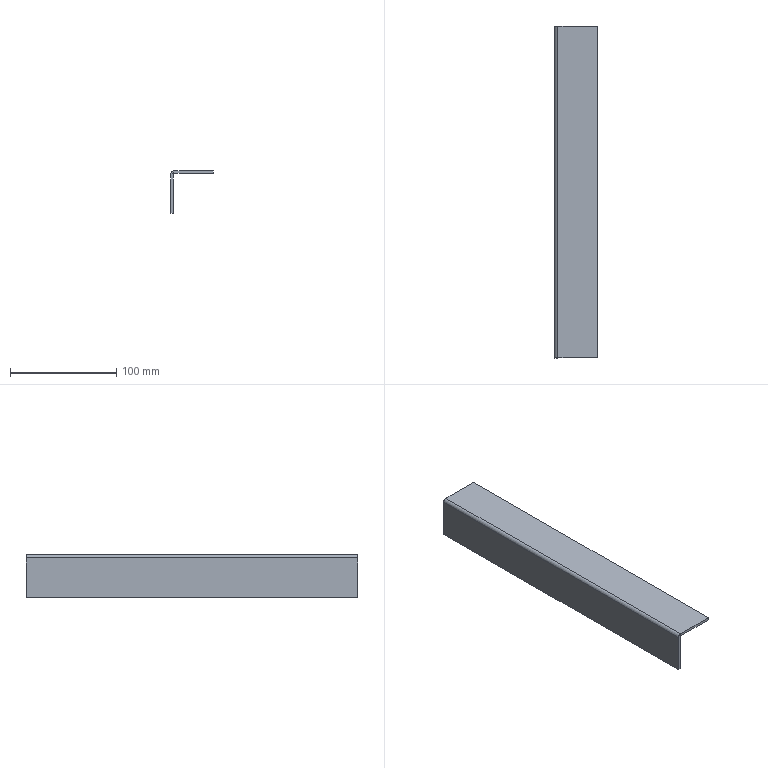Component | SolidWorks | BottomFrameAssembly2-1_CabinetDepthBeam-2 | 1 solid | 14 faces | box 40 x 313 x 40 mm | volume 60056 mm3 | plane 12 | cylinder 2 | commonest cylinder face diameters 1 x1 6 x1
STEP:
#1=CARTESIAN_POINT('',(-5.573,-6.388,66.81));
#2=VERTEX_POINT('',#1);
#3=CARTESIAN_POINT('',(-5.672,-6.388,66.81));
#4=VERTEX_POINT('',#3);
#5=CARTESIAN_POINT('',(-5.573,-6.388,66.81));
#6=DIRECTION('',(-1.,-0.,0.));
#7=VECTOR('',#6,39.37);
#8=LINE('',#5,#7);
#9=EDGE_CURVE('',#2,#4,#8,.T.);
#10=ORIENTED_EDGE('',*,*,#9,.F.);
#11=CARTESIAN_POINT('',(-5.554,-6.388,66.83));
#12=VERTEX_POINT('',#11);
#13=CARTESIAN_POINT('',(-5.554,-6.388,66.81));
#14=DIRECTION('',(0.,-1.,0.));
#15=DIRECTION('',(1.,0.,0.));
#16=AXIS2_PLACEMENT_3D('',#13,#14,#15);
#17=CIRCLE('',#16,0.01969);
#18=EDGE_CURVE('',#12,#2,#17,.T.);
#19=ORIENTED_EDGE('',*,*,#18,.F.);
#20=CARTESIAN_POINT('',(-5.554,-6.388,66.928));
#21=VERTEX_POINT('',#20);
#22=CARTESIAN_POINT('',(-5.554,-6.388,66.928));
#23=DIRECTION('',(0.,-0.,-1.));
#24=VECTOR('',#23,39.37);
#25=LINE('',#22,#24);
#26=EDGE_CURVE('',#21,#12,#25,.T.);
#27=ORIENTED_EDGE('',*,*,#26,.F.);
#28=CARTESIAN_POINT('',(-5.554,-6.388,66.81));
#29=DIRECTION('',(0.,-1.,0.));
#30=DIRECTION('',(-1.,-0.,0.));
#31=AXIS2_PLACEMENT_3D('',#28,#29,#30);
#32=CIRCLE('',#31,0.1181);
#33=EDGE_CURVE('',#21,#4,#32,.T.);
#34=ORIENTED_EDGE('',*,*,#33,.T.);
#35=EDGE_LOOP('',(#10,#19,#27,#34));
#36=FACE_OUTER_BOUND('',#35,.T.);
#37=CARTESIAN_POINT('',(-5.573,-6.388,66.81));
#38=DIRECTION('',(0.,-1.,0.));
#39=DIRECTION('',(-1.,-0.,0.));
#40=AXIS2_PLACEMENT_3D('',#37,#38,#39);
#41=PLANE('',#40);
#42=ADVANCED_FACE('',(#36),#41,.T.);
#43=CARTESIAN_POINT('',(-5.573,-6.388,65.354));
#44=VERTEX_POINT('',#43);
#45=CARTESIAN_POINT('',(-5.573,-6.388,66.83));
#46=DIRECTION('',(0.,-0.,-1.));
#47=VECTOR('',#46,39.37);
#48=LINE('',#45,#47);
#49=EDGE_CURVE('',#2,#44,#48,.T.);
#50=ORIENTED_EDGE('',*,*,#49,.F.);
#51=ORIENTED_EDGE('',*,*,#9,.T.);
#52=CARTESIAN_POINT('',(-5.672,-6.388,65.354));
#53=VERTEX_POINT('',#52);
#54=CARTESIAN_POINT('',(-5.672,-6.388,66.83));
#55=DIRECTION('',(0.,-0.,-1.));
#56=VECTOR('',#55,39.37);
#57=LINE('',#54,#56);
#58=EDGE_CURVE('',#4,#53,#57,.T.);
#59=ORIENTED_EDGE('',*,*,#58,.T.);
#60=CARTESIAN_POINT('',(-5.573,-6.388,65.354));
#61=DIRECTION('',(-1.,-0.,0.));
#62=VECTOR('',#61,39.37);
#63=LINE('',#60,#62);
#64=EDGE_CURVE('',#44,#53,#63,.T.);
#65=ORIENTED_EDGE('',*,*,#64,.F.);
#66=EDGE_LOOP('',(#50,#51,#59,#65));
#67=FACE_OUTER_BOUND('',#66,.T.);
#68=CARTESIAN_POINT('',(-5.554,-6.388,66.928));
#69=DIRECTION('',(0.,-1.,0.));
#70=DIRECTION('',(-1.,-0.,0.));
#71=AXIS2_PLACEMENT_3D('',#68,#69,#70);
#72=PLANE('',#71);
#73=ADVANCED_FACE('',(#67),#72,.T.);
#74=CARTESIAN_POINT('',(-5.554,5.935,66.83));
#75=VERTEX_POINT('',#74);
#76=CARTESIAN_POINT('',(-5.554,5.935,66.928));
#77=VERTEX_POINT('',#76);
#78=CARTESIAN_POINT('',(-5.554,5.935,66.83));
#79=DIRECTION('',(-0.,0.,1.));
#80=VECTOR('',#79,39.37);
#81=LINE('',#78,#80);
#82=EDGE_CURVE('',#75,#77,#81,.T.);
#83=ORIENTED_EDGE('',*,*,#82,.F.);
#84=CARTESIAN_POINT('',(-5.573,5.935,66.81));
#85=VERTEX_POINT('',#84);
#86=CARTESIAN_POINT('',(-5.554,5.935,66.81));
#87=DIRECTION('',(0.,-1.,0.));
#88=DIRECTION('',(1.,0.,0.));
#89=AXIS2_PLACEMENT_3D('',#86,#87,#88);
#90=CIRCLE('',#89,0.01969);
#91=EDGE_CURVE('',#75,#85,#90,.T.);
#92=ORIENTED_EDGE('',*,*,#91,.T.);
#93=CARTESIAN_POINT('',(-5.672,5.935,66.81));
#94=VERTEX_POINT('',#93);
#95=CARTESIAN_POINT('',(-5.672,5.935,66.81));
#96=DIRECTION('',(1.,0.,-0.));
#97=VECTOR('',#96,39.37);
#98=LINE('',#95,#97);
#99=EDGE_CURVE('',#94,#85,#98,.T.);
#100=ORIENTED_EDGE('',*,*,#99,.F.);
#101=CARTESIAN_POINT('',(-5.554,5.935,66.81));
#102=DIRECTION('',(0.,-1.,0.));
#103=DIRECTION('',(-1.,-0.,0.));
#104=AXIS2_PLACEMENT_3D('',#101,#102,#103);
#105=CIRCLE('',#104,0.1181);
#106=EDGE_CURVE('',#77,#94,#105,.T.);
#107=ORIENTED_EDGE('',*,*,#106,.F.);
#108=EDGE_LOOP('',(#83,#92,#100,#107));
#109=FACE_OUTER_BOUND('',#108,.T.);
#110=CARTESIAN_POINT('',(-5.554,5.935,66.83));
#111=DIRECTION('',(-0.,1.,-0.));
#112=DIRECTION('',(1.,0.,-0.));
#113=AXIS2_PLACEMENT_3D('',#110,#111,#112);
#114=PLANE('',#113);
#115=ADVANCED_FACE('',(#109),#114,.T.);
#116=CARTESIAN_POINT('',(-4.097,5.935,66.83));
#117=VERTEX_POINT('',#116);
#118=CARTESIAN_POINT('',(-4.097,5.935,66.83));
#119=DIRECTION('',(-1.,-0.,0.));
#120=VECTOR('',#119,39.37);
#121=LINE('',#118,#120);
#122=EDGE_CURVE('',#117,#75,#121,.T.);
#123=ORIENTED_EDGE('',*,*,#122,.T.);
#124=ORIENTED_EDGE('',*,*,#82,.T.);
#125=CARTESIAN_POINT('',(-4.097,5.935,66.928));
#126=VERTEX_POINT('',#125);
#127=CARTESIAN_POINT('',(-4.097,5.935,66.928));
#128=DIRECTION('',(-1.,-0.,0.));
#129=VECTOR('',#128,39.37);
#130=LINE('',#127,#129);
#131=EDGE_CURVE('',#126,#77,#130,.T.);
#132=ORIENTED_EDGE('',*,*,#131,.F.);
#133=CARTESIAN_POINT('',(-4.097,5.935,66.928));
#134=DIRECTION('',(0.,-0.,-1.));
#135=VECTOR('',#134,39.37);
#136=LINE('',#133,#135);
#137=EDGE_CURVE('',#126,#117,#136,.T.);
#138=ORIENTED_EDGE('',*,*,#137,.T.);
#139=EDGE_LOOP('',(#123,#124,#132,#138));
#140=FACE_OUTER_BOUND('',#139,.T.);
#141=CARTESIAN_POINT('',(-5.672,5.935,66.81));
#142=DIRECTION('',(-0.,1.,-0.));
#143=DIRECTION('',(1.,0.,-0.));
#144=AXIS2_PLACEMENT_3D('',#141,#142,#143);
#145=PLANE('',#144);
#146=ADVANCED_FACE('',(#140),#145,.T.);
#147=CARTESIAN_POINT('',(-5.672,5.935,65.354));
#148=VERTEX_POINT('',#147);
#149=CARTESIAN_POINT('',(-5.672,5.935,66.83));
#150=DIRECTION('',(0.,-0.,-1.));
#151=VECTOR('',#150,39.37);
#152=LINE('',#149,#151);
#153=EDGE_CURVE('',#94,#148,#152,.T.);
#154=ORIENTED_EDGE('',*,*,#153,.T.);
#155=CARTESIAN_POINT('',(-5.672,-6.388,65.354));
#156=DIRECTION('',(-0.,1.,-0.));
#157=VECTOR('',#156,39.37);
#158=LINE('',#155,#157);
#159=EDGE_CURVE('',#53,#148,#158,.T.);
#160=ORIENTED_EDGE('',*,*,#159,.F.);
#161=ORIENTED_EDGE('',*,*,#58,.F.);
#162=CARTESIAN_POINT('',(-5.672,-6.388,66.81));
#163=DIRECTION('',(-0.,1.,-0.));
#164=VECTOR('',#163,39.37);
#165=LINE('',#162,#164);
#166=EDGE_CURVE('',#4,#94,#165,.T.);
#167=ORIENTED_EDGE('',*,*,#166,.T.);
#168=EDGE_LOOP('',(#154,#160,#161,#167));
#169=FACE_OUTER_BOUND('',#168,.T.);
#170=CARTESIAN_POINT('',(-5.672,-6.388,66.83));
#171=DIRECTION('',(1.,0.,-0.));
#172=DIRECTION('',(0.,-1.,0.));
#173=AXIS2_PLACEMENT_3D('',#170,#171,#172);
#174=PLANE('',#173);
#175=ADVANCED_FACE('',(#169),#174,.F.);
#176=CARTESIAN_POINT('',(-5.573,5.935,65.354));
#177=VERTEX_POINT('',#176);
#178=CARTESIAN_POINT('',(-5.573,5.935,65.354));
#179=DIRECTION('',(-1.,-0.,0.));
#180=VECTOR('',#179,39.37);
#181=LINE('',#178,#180);
#182=EDGE_CURVE('',#177,#148,#181,.T.);
#183=ORIENTED_EDGE('',*,*,#182,.F.);
#184=CARTESIAN_POINT('',(-5.573,-6.388,65.354));
#185=DIRECTION('',(-0.,1.,-0.));
#186=VECTOR('',#185,39.37);
#187=LINE('',#184,#186);
#188=EDGE_CURVE('',#44,#177,#187,.T.);
#189=ORIENTED_EDGE('',*,*,#188,.F.);
#190=ORIENTED_EDGE('',*,*,#64,.T.);
#191=ORIENTED_EDGE('',*,*,#159,.T.);
#192=EDGE_LOOP('',(#183,#189,#190,#191));
#193=FACE_OUTER_BOUND('',#192,.T.);
#194=CARTESIAN_POINT('',(-5.573,-6.388,65.354));
#195=DIRECTION('',(0.,-0.,-1.));
#196=DIRECTION('',(0.,-1.,0.));
#197=AXIS2_PLACEMENT_3D('',#194,#195,#196);
#198=PLANE('',#197);
#199=ADVANCED_FACE('',(#193),#198,.T.);
#200=CARTESIAN_POINT('',(-5.573,5.935,66.83));
#201=DIRECTION('',(0.,-0.,-1.));
#202=VECTOR('',#201,39.37);
#203=LINE('',#200,#202);
#204=EDGE_CURVE('',#85,#177,#203,.T.);
#205=ORIENTED_EDGE('',*,*,#204,.F.);
#206=CARTESIAN_POINT('',(-5.573,-6.388,66.81));
#207=DIRECTION('',(-0.,1.,-0.));
#208=VECTOR('',#207,39.37);
#209=LINE('',#206,#208);
#210=EDGE_CURVE('',#2,#85,#209,.T.);
#211=ORIENTED_EDGE('',*,*,#210,.F.);
#212=ORIENTED_EDGE('',*,*,#49,.T.);
#213=ORIENTED_EDGE('',*,*,#188,.T.);
#214=EDGE_LOOP('',(#205,#211,#212,#213));
#215=FACE_OUTER_BOUND('',#214,.T.);
#216=CARTESIAN_POINT('',(-5.573,-6.388,66.83));
#217=DIRECTION('',(1.,0.,-0.));
#218=DIRECTION('',(0.,-1.,0.));
#219=AXIS2_PLACEMENT_3D('',#216,#217,#218);
#220=PLANE('',#219);
#221=ADVANCED_FACE('',(#215),#220,.T.);
#222=ORIENTED_EDGE('',*,*,#91,.F.);
#223=CARTESIAN_POINT('',(-5.554,-6.388,66.83));
#224=DIRECTION('',(-0.,1.,-0.));
#225=VECTOR('',#224,39.37);
#226=LINE('',#223,#225);
#227=EDGE_CURVE('',#12,#75,#226,.T.);
#228=ORIENTED_EDGE('',*,*,#227,.F.);
#229=ORIENTED_EDGE('',*,*,#18,.T.);
#230=ORIENTED_EDGE('',*,*,#210,.T.);
#231=EDGE_LOOP('',(#222,#228,#229,#230));
#232=FACE_OUTER_BOUND('',#231,.T.);
#233=CARTESIAN_POINT('',(-5.554,-6.388,66.81));
#234=DIRECTION('',(-0.,1.,-0.));
#235=DIRECTION('',(1.,0.,0.));
#236=AXIS2_PLACEMENT_3D('',#233,#234,#235);
#237=CYLINDRICAL_SURFACE('',#236,0.01969);
#238=ADVANCED_FACE('',(#232),#237,.F.);
#239=ORIENTED_EDGE('',*,*,#122,.F.);
#240=CARTESIAN_POINT('',(-4.097,-6.388,66.83));
#241=VERTEX_POINT('',#240);
#242=CARTESIAN_POINT('',(-4.097,-6.388,66.83));
#243=DIRECTION('',(-0.,1.,-0.));
#244=VECTOR('',#243,39.37);
#245=LINE('',#242,#244);
#246=EDGE_CURVE('',#241,#117,#245,.T.);
#247=ORIENTED_EDGE('',*,*,#246,.F.);
#248=CARTESIAN_POINT('',(-4.097,-6.388,66.83));
#249=DIRECTION('',(-1.,-0.,0.));
#250=VECTOR('',#249,39.37);
#251=LINE('',#248,#250);
#252=EDGE_CURVE('',#241,#12,#251,.T.);
#253=ORIENTED_EDGE('',*,*,#252,.T.);
#254=ORIENTED_EDGE('',*,*,#227,.T.);
#255=EDGE_LOOP('',(#239,#247,#253,#254));
#256=FACE_OUTER_BOUND('',#255,.T.);
#257=CARTESIAN_POINT('',(-4.097,-6.388,66.83));
#258=DIRECTION('',(0.,-0.,-1.));
#259=DIRECTION('',(0.,-1.,0.));
#260=AXIS2_PLACEMENT_3D('',#257,#258,#259);
#261=PLANE('',#260);
#262=ADVANCED_FACE('',(#256),#261,.T.);
#263=ORIENTED_EDGE('',*,*,#137,.F.);
#264=CARTESIAN_POINT('',(-4.097,-6.388,66.928));
#265=VERTEX_POINT('',#264);
#266=CARTESIAN_POINT('',(-4.097,-6.388,66.928));
#267=DIRECTION('',(-0.,1.,-0.));
#268=VECTOR('',#267,39.37);
#269=LINE('',#266,#268);
#270=EDGE_CURVE('',#265,#126,#269,.T.);
#271=ORIENTED_EDGE('',*,*,#270,.F.);
#272=CARTESIAN_POINT('',(-4.097,-6.388,66.928));
#273=DIRECTION('',(0.,-0.,-1.));
#274=VECTOR('',#273,39.37);
#275=LINE('',#272,#274);
#276=EDGE_CURVE('',#265,#241,#275,.T.);
#277=ORIENTED_EDGE('',*,*,#276,.T.);
#278=ORIENTED_EDGE('',*,*,#246,.T.);
#279=EDGE_LOOP('',(#263,#271,#277,#278));
#280=FACE_OUTER_BOUND('',#279,.T.);
#281=CARTESIAN_POINT('',(-4.097,-6.388,66.928));
#282=DIRECTION('',(1.,0.,-0.));
#283=DIRECTION('',(0.,-1.,0.));
#284=AXIS2_PLACEMENT_3D('',#281,#282,#283);
#285=PLANE('',#284);
#286=ADVANCED_FACE('',(#280),#285,.T.);
#287=ORIENTED_EDGE('',*,*,#131,.T.);
#288=CARTESIAN_POINT('',(-5.554,-6.388,66.928));
#289=DIRECTION('',(-0.,1.,-0.));
#290=VECTOR('',#289,39.37);
#291=LINE('',#288,#290);
#292=EDGE_CURVE('',#21,#77,#291,.T.);
#293=ORIENTED_EDGE('',*,*,#292,.F.);
#294=CARTESIAN_POINT('',(-4.097,-6.388,66.928));
#295=DIRECTION('',(-1.,-0.,0.));
#296=VECTOR('',#295,39.37);
#297=LINE('',#294,#296);
#298=EDGE_CURVE('',#265,#21,#297,.T.);
#299=ORIENTED_EDGE('',*,*,#298,.F.);
#300=ORIENTED_EDGE('',*,*,#270,.T.);
#301=EDGE_LOOP('',(#287,#293,#299,#300));
#302=FACE_OUTER_BOUND('',#301,.T.);
#303=CARTESIAN_POINT('',(-4.097,-6.388,66.928));
#304=DIRECTION('',(0.,-0.,-1.));
#305=DIRECTION('',(0.,-1.,0.));
#306=AXIS2_PLACEMENT_3D('',#303,#304,#305);
#307=PLANE('',#306);
#308=ADVANCED_FACE('',(#302),#307,.F.);
#309=ORIENTED_EDGE('',*,*,#106,.T.);
#310=ORIENTED_EDGE('',*,*,#166,.F.);
#311=ORIENTED_EDGE('',*,*,#33,.F.);
#312=ORIENTED_EDGE('',*,*,#292,.T.);
#313=EDGE_LOOP('',(#309,#310,#311,#312));
#314=FACE_OUTER_BOUND('',#313,.T.);
#315=CARTESIAN_POINT('',(-5.554,-6.388,66.81));
#316=DIRECTION('',(-0.,1.,-0.));
#317=DIRECTION('',(1.,0.,0.));
#318=AXIS2_PLACEMENT_3D('',#315,#316,#317);
#319=CYLINDRICAL_SURFACE('',#318,0.1181);
#320=ADVANCED_FACE('',(#314),#319,.T.);
#321=ORIENTED_EDGE('',*,*,#298,.T.);
#322=ORIENTED_EDGE('',*,*,#26,.T.);
#323=ORIENTED_EDGE('',*,*,#252,.F.);
#324=ORIENTED_EDGE('',*,*,#276,.F.);
#325=EDGE_LOOP('',(#321,#322,#323,#324));
#326=FACE_OUTER_BOUND('',#325,.T.);
#327=CARTESIAN_POINT('',(-5.554,-6.388,66.81));
#328=DIRECTION('',(-0.,1.,-0.));
#329=DIRECTION('',(1.,0.,-0.));
#330=AXIS2_PLACEMENT_3D('',#327,#328,#329);
#331=PLANE('',#330);
#332=ADVANCED_FACE('',(#326),#331,.F.);
#333=ORIENTED_EDGE('',*,*,#153,.F.);
#334=ORIENTED_EDGE('',*,*,#99,.T.);
#335=ORIENTED_EDGE('',*,*,#204,.T.);
#336=ORIENTED_EDGE('',*,*,#182,.T.);
#337=EDGE_LOOP('',(#333,#334,#335,#336));
#338=FACE_OUTER_BOUND('',#337,.T.);
#339=CARTESIAN_POINT('',(-5.554,5.935,66.81));
#340=DIRECTION('',(-0.,1.,-0.));
#341=DIRECTION('',(1.,0.,-0.));
#342=AXIS2_PLACEMENT_3D('',#339,#340,#341);
#343=PLANE('',#342);
#344=ADVANCED_FACE('',(#338),#343,.T.);
#345=CLOSED_SHELL('',(#42,#73,#115,#146,#175,#199,#221,#238,#262,#286,#308,#320,#332,#344));
#346=MANIFOLD_SOLID_BREP('',#345);
#347=CARTESIAN_POINT('',(0.,0.,0.));
#348=DIRECTION('',(0.,0.,1.));
#349=DIRECTION('',(1.,0.,0.));
#350=AXIS2_PLACEMENT_3D('',#347,#348,#349);
#351=(LENGTH_UNIT()NAMED_UNIT(*)SI_UNIT($,.METRE.));
#352=LENGTH_MEASURE_WITH_UNIT(LENGTH_MEASURE(0.0254),#351);
#353=DIMENSIONAL_EXPONENTS(1.,0.,0.,0.,0.,0.,0.);
#354=(CONVERSION_BASED_UNIT('',#352)LENGTH_UNIT()NAMED_UNIT(#353));
#355=UNCERTAINTY_MEASURE_WITH_UNIT(LENGTH_MEASURE(0.00001),#354,'','');
#356=(NAMED_UNIT(*)PLANE_ANGLE_UNIT()SI_UNIT($,.RADIAN.));
#357=(NAMED_UNIT(*)SI_UNIT($,.STERADIAN.)SOLID_ANGLE_UNIT());
#358=(GEOMETRIC_REPRESENTATION_CONTEXT(3)GLOBAL_UNCERTAINTY_ASSIGNED_CONTEXT((#355))GLOBAL_UNIT_ASSIGNED_CONTEXT((#354,#356,#357))REPRESENTATION_CONTEXT('',''));
#359=ADVANCED_BREP_SHAPE_REPRESENTATION('',(#346,#350),#358);
#360=COLOUR_RGB('',0.7922,0.8196,0.9333);
#361=FILL_AREA_STYLE_COLOUR('',#360);
#362=FILL_AREA_STYLE('',(#361));
#363=SURFACE_STYLE_FILL_AREA(#362);
#364=SURFACE_SIDE_STYLE('',(#363));
#365=SURFACE_STYLE_USAGE(.BOTH.,#364);
#366=PRESENTATION_STYLE_ASSIGNMENT((#365));
#367=STYLED_ITEM('',(#366),#346);
#368=(LENGTH_UNIT()NAMED_UNIT(*)SI_UNIT($,.METRE.));
#369=LENGTH_MEASURE_WITH_UNIT(LENGTH_MEASURE(0.0254),#368);
#370=DIMENSIONAL_EXPONENTS(1.,0.,0.,0.,0.,0.,0.);
#371=(CONVERSION_BASED_UNIT('',#369)LENGTH_UNIT()NAMED_UNIT(#370));
#372=UNCERTAINTY_MEASURE_WITH_UNIT(LENGTH_MEASURE(0.00001),#371,'','');
#373=(NAMED_UNIT(*)PLANE_ANGLE_UNIT()SI_UNIT($,.RADIAN.));
#374=(NAMED_UNIT(*)SI_UNIT($,.STERADIAN.)SOLID_ANGLE_UNIT());
#375=(GEOMETRIC_REPRESENTATION_CONTEXT(3)GLOBAL_UNCERTAINTY_ASSIGNED_CONTEXT((#372))GLOBAL_UNIT_ASSIGNED_CONTEXT((#371,#373,#374))REPRESENTATION_CONTEXT('',''));
#376=MECHANICAL_DESIGN_GEOMETRIC_PRESENTATION_REPRESENTATION('',(#367),#375);
#377=PRESENTATION_LAYER_ASSIGNMENT('','',(#367));